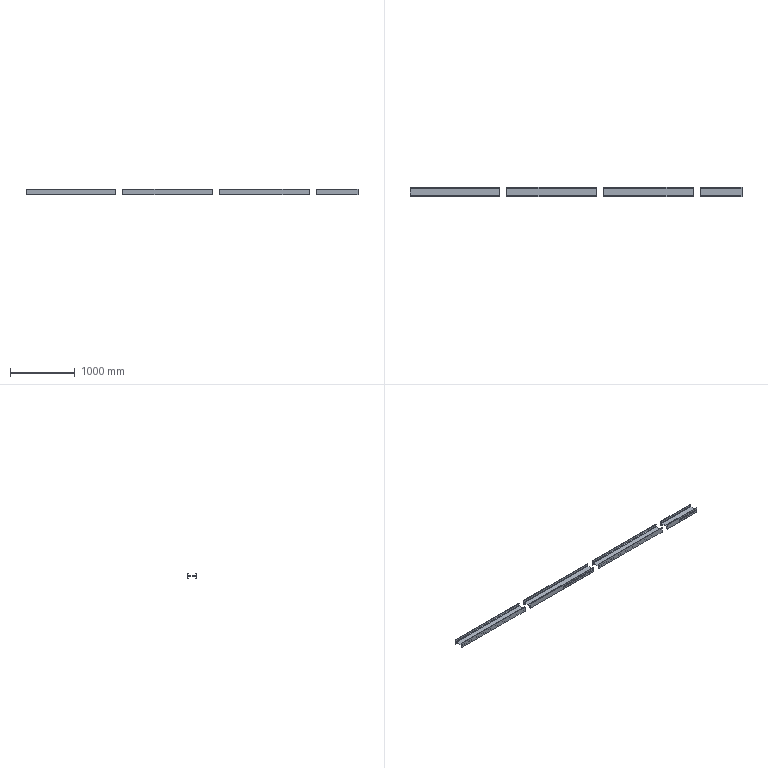Component | NX | P5 | 4 solids | 72 faces | volume 10420871 mm3 | plane 56 | cylinder 16 | commonest cylinder face diameters 15 x16